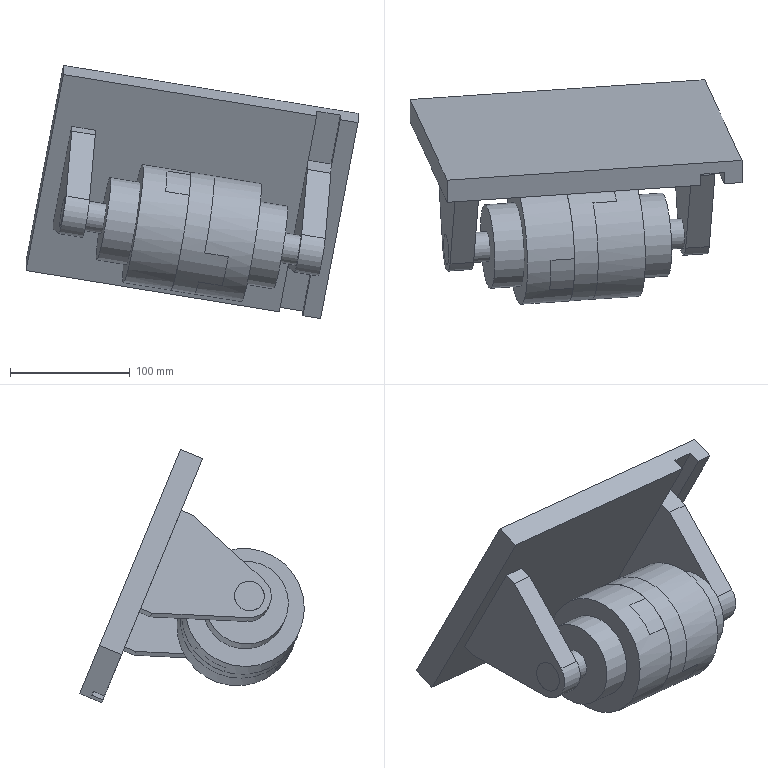Assembly | NX | mm | 5 component files | 8 solids | 83 faces | box 277.46 x 187.76 x 211.59 mm | volume 1916205 mm3 | plane 65 | cylinder 18 | commonest cylinder face diameters 100 x5 50 x5 25 x4 36.69 x2 70 x2
Bill of materials:
unnamed part 1 | 2 |  | Stepped, coaxial cylindrical body with three diameters: a small pin, a middle collar, and a larger hub. The end face of the hub has two rectangular slots on opposite sides and a shallow central circular recess or bore.
unnamed part 2 | 1 |  | Thin flat rectangular plate with a single tapered lug standing perpendicular to it near one edge. The lug has a rounded tip with a round through-hole. One edge of the plate has a small rectangular step or notch.
unnamed part 3 | 1 |  | Annular disc with a central through-hole. Each face has a pair of rectangular lugs on opposite sides; the pair on one face is turned about 90 degrees from the pair on the other, giving a cross-shaped pattern.
unnamed part 4 | 1 |  | Flat plate shaped roughly like a trapezoid or triangle. It narrows to a rounded end with a circular through-hole, and the wide end has two angled cut corners.
Mates:
1. touch align | 3 1 face | 2 1 face
2. touch align | 3 1 edge | 2 1 edge
3. touch align | 2 1 face | 1 1 face
4. touch align | 2 2 face | 4 1 face
5. touch align | 4 1 face | 1 1 face
6. touch align | 4 1 edge | 1 1 face
7. touch align | 2 2 edge | 4 1 edge
8. fix | 1 1 component
9. parallel | 4 1 face | 1 1 face